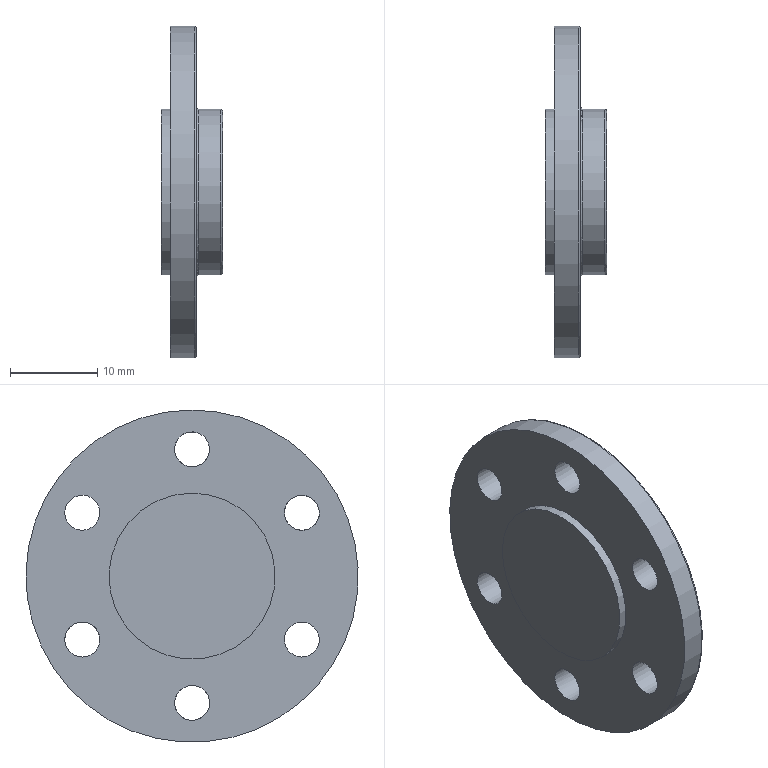Component | NX | OUTER_END_COVER | 1 solid | 16 faces | volume 4309 mm3 | cylinder 9 | plane 4 | torus 3 | commonest cylinder face diameters 4 x6 19 x2 38 x1